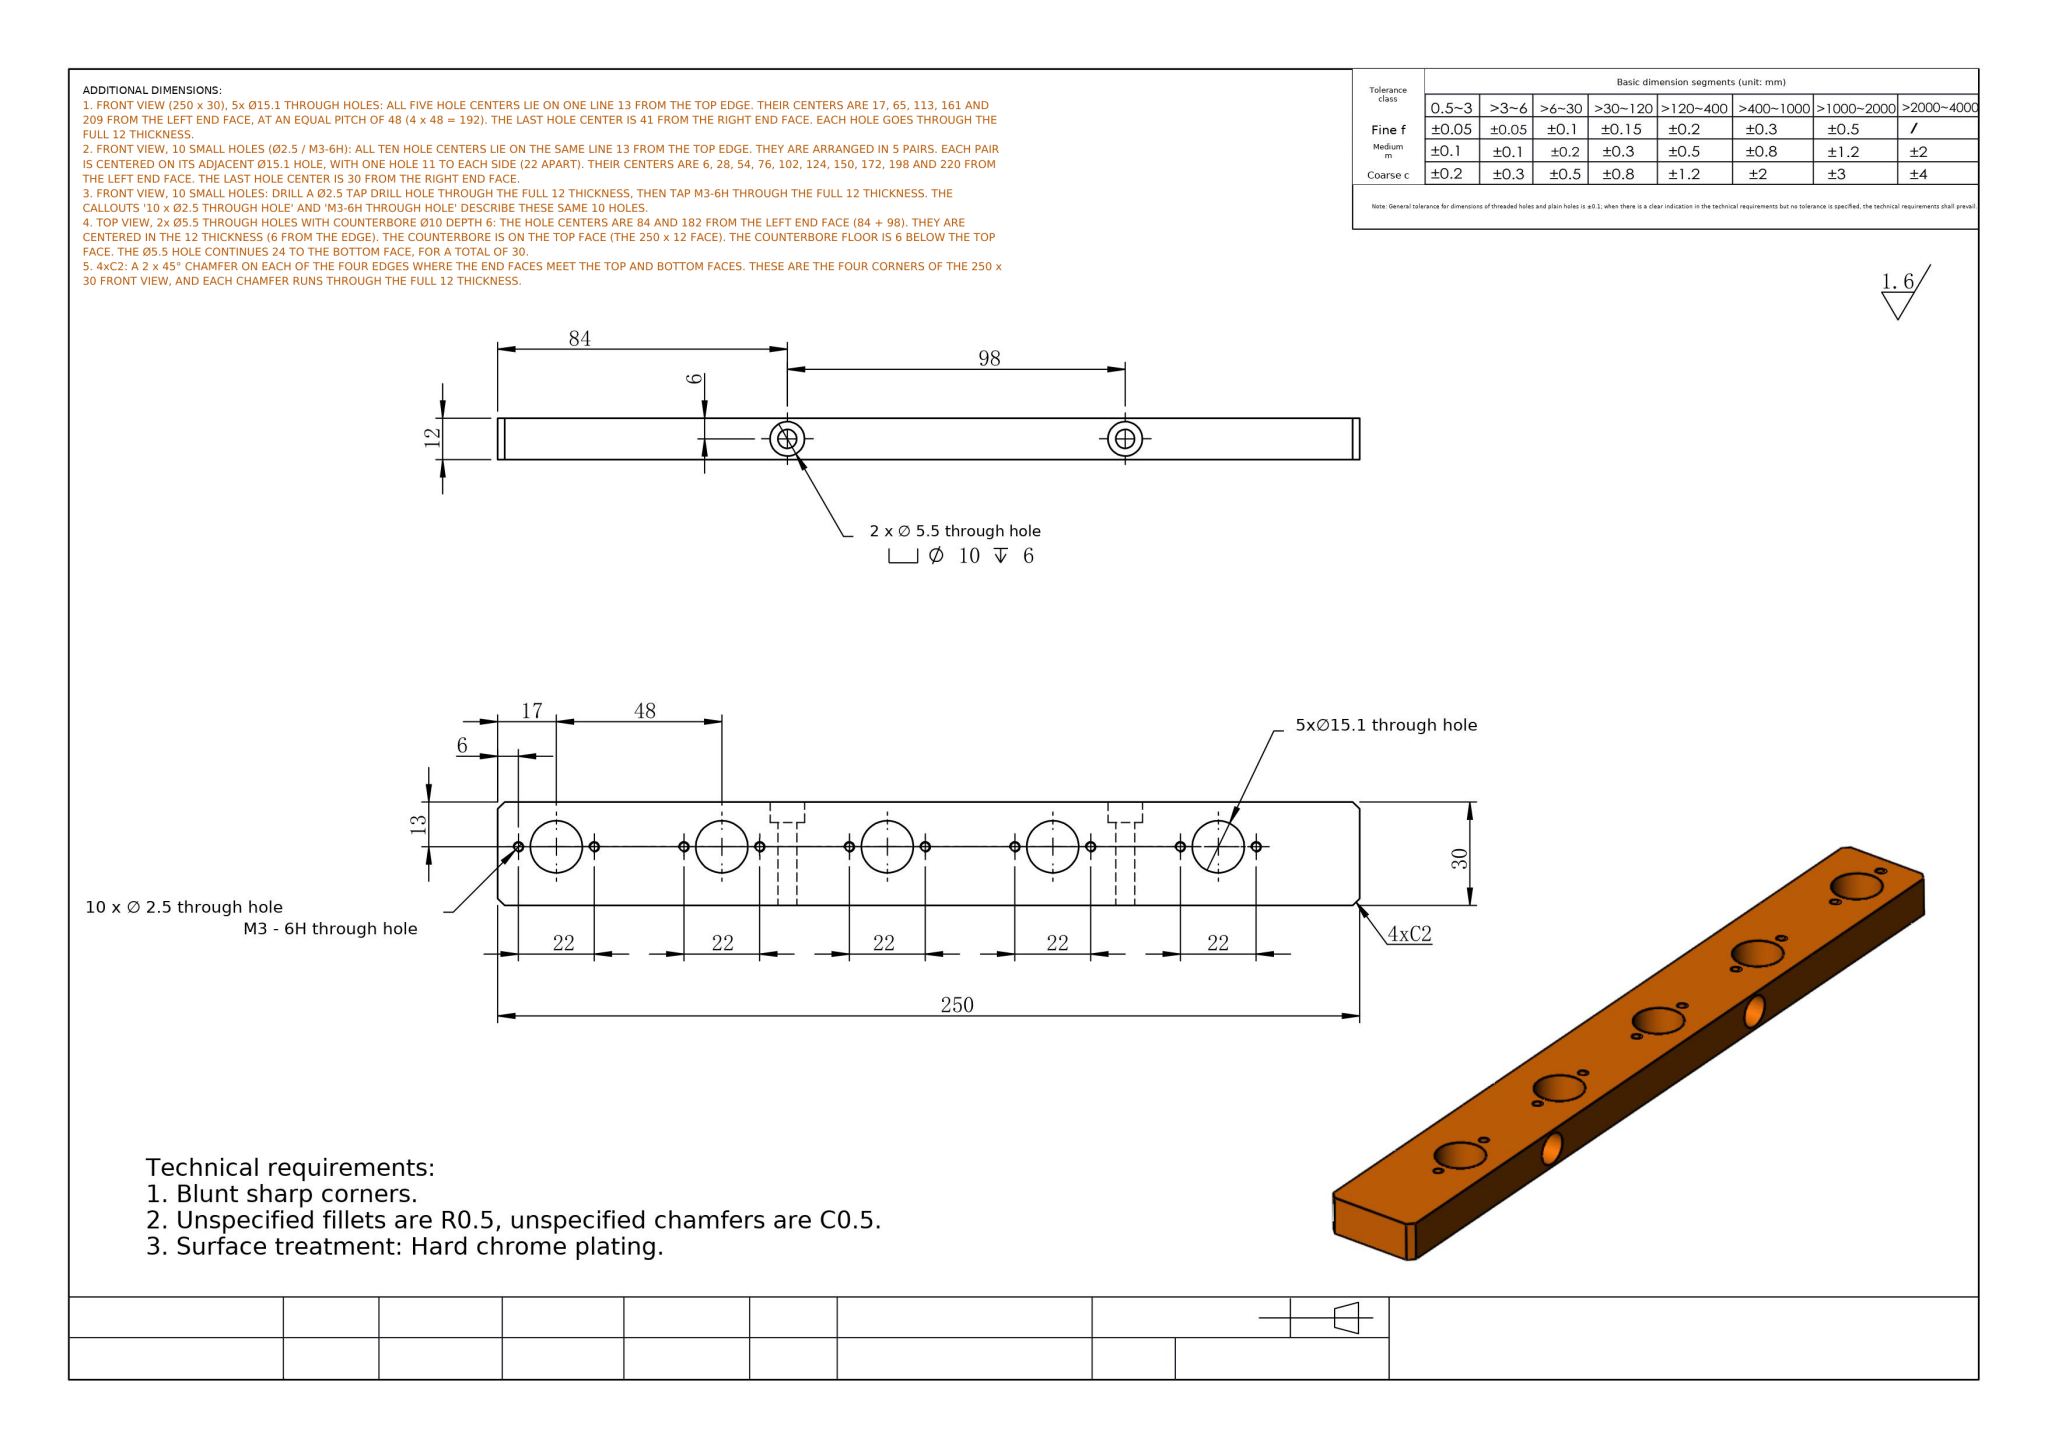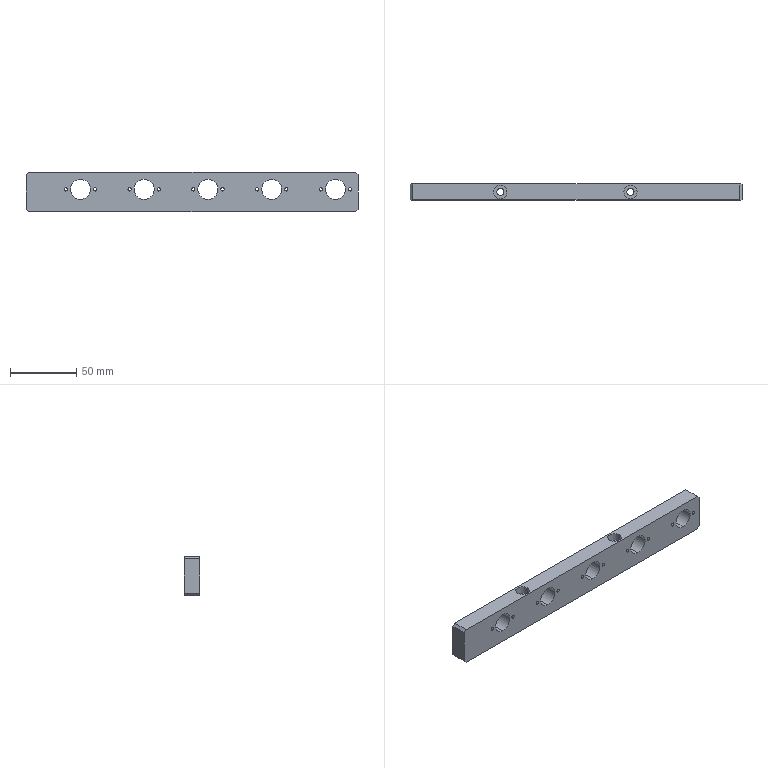Part | NX | mm | Rounded Corner Ten-Bore Mounting Rail | 1 solid | 50 faces | box 250 x 12 x 30 mm | volume 76487 mm3 | cylinder 38 | plane 12 | commonest cylinder face diameters 2.5 x20 15.1 x10 10 x4 5.5 x4